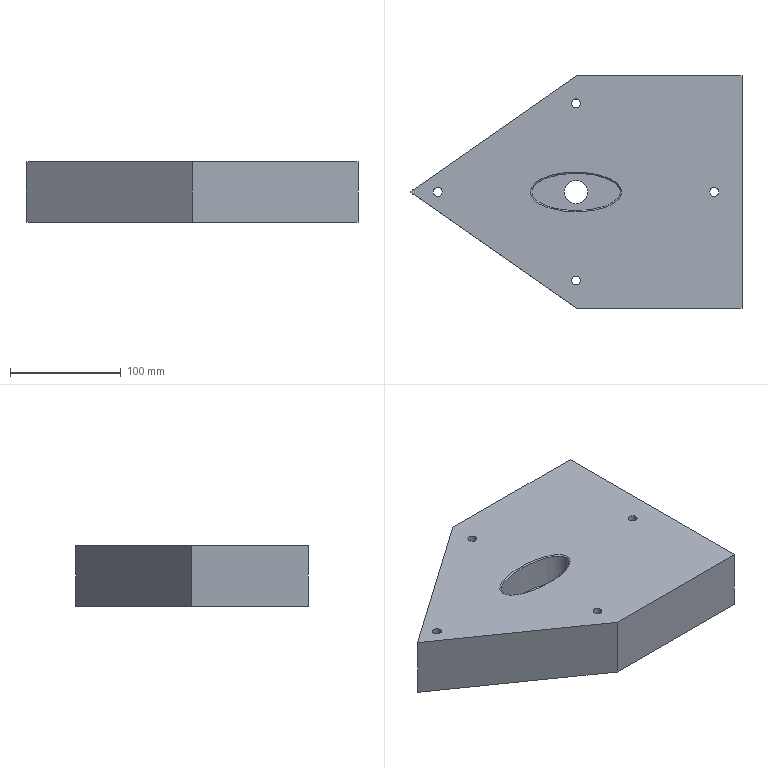Component | NX | TRIM_PUNCH_DIE | 1 solid | 23 faces | volume 2503069 mm3 | plane 12 | cylinder 9 | other 1 | spline 1 | commonest cylinder face diameters 8.06 x4 12.06 x4 21 x1